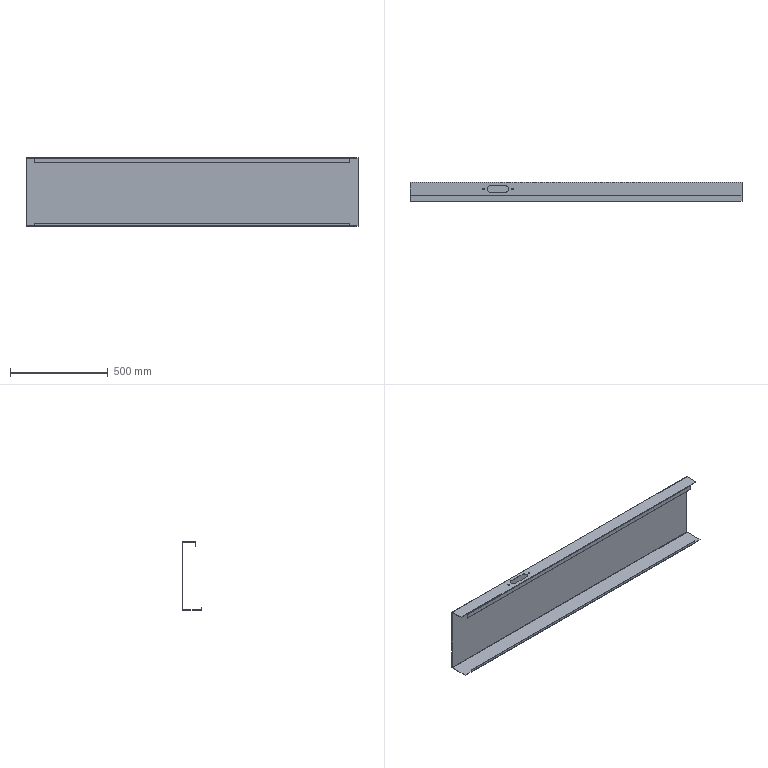Component | SolidWorks | RightSidePlate-1 | 1 solid | 46 faces | volume 1851503 mm3 | plane 32 | cylinder 14 | commonest cylinder face diameters 9 x4 6 x4 2 x4 32 x2